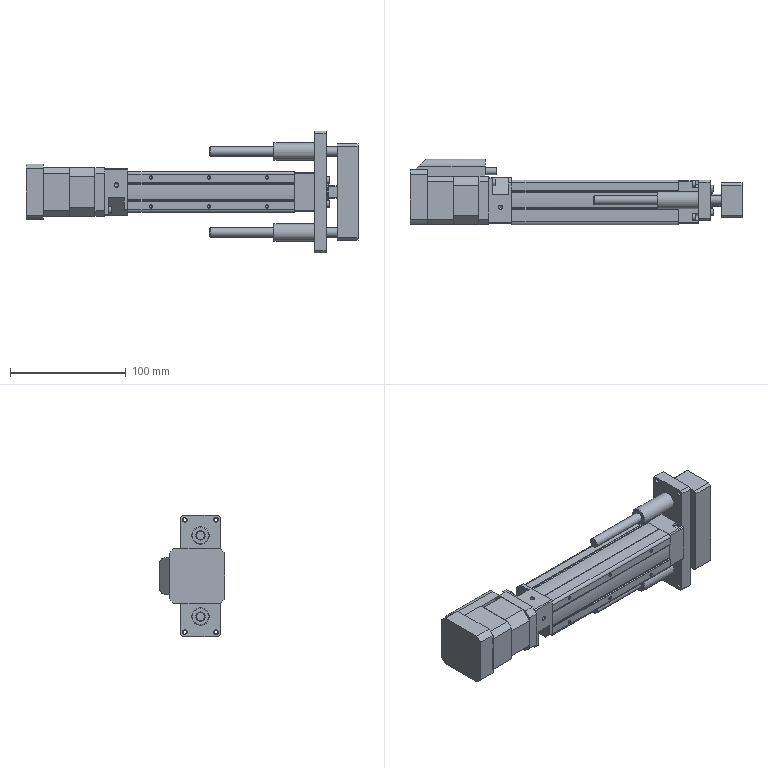Assembly | NX | mm | 5 component files | 5 solids | 347 faces | box 286.5 x 56.5 x 105 mm | volume 481263 mm3 | plane 181 | cylinder 88 | cone 78 | commonest cylinder face diameters 3.242 x16 5.5 x10 2.459 x10 0.4 x8 2 x8 6 x7 8 x6 5 x4
Bill of materials:
unnamed part 1 | 1 |  | Long prismatic body with a roughly square cross-section. One end has a larger stepped block with chamfered corners; the other end has an end cap with a large circular bore and small holes around it. It looks like a linear actuator or slide-type unit, but this is not confirmed.
unnamed part 2 | 1 |  | Rectangular block with chamfered corners. Two long parallel cylindrical rods of the same size stick out from one face. The opposite face has a central through-hole and eight small holes in a 2 x 4 pattern.
unnamed part 3 | 1 |  | Hexagonal nut shape: a flat hexagonal prism with a central circular bore and chamfered edges on both faces.
unnamed part 4 | 1 |  | Stepped cylindrical shaft or pin. It has a long, larger-diameter main body, a short section with flats, a narrow neck or groove, and a smaller cylindrical end pin with a chamfered tip.
unnamed part 5 | 1 |  | Rectangular plate with chamfered corners. Two large cylindrical bosses stick out from one face, and two short cylindrical pins stick out from the opposite face. The plate has a large central hole, two medium holes, four small corner holes and several small features around the central hole.
Mates:
1. fix | Slide_Rail 1 component
2. fix | Fixed_Nut 1 component
3. fix | Slide_Table 1 component
4. fix | Push_Rod 1 component
5. fix | Slide_Rail_Cyl_Body 1 component